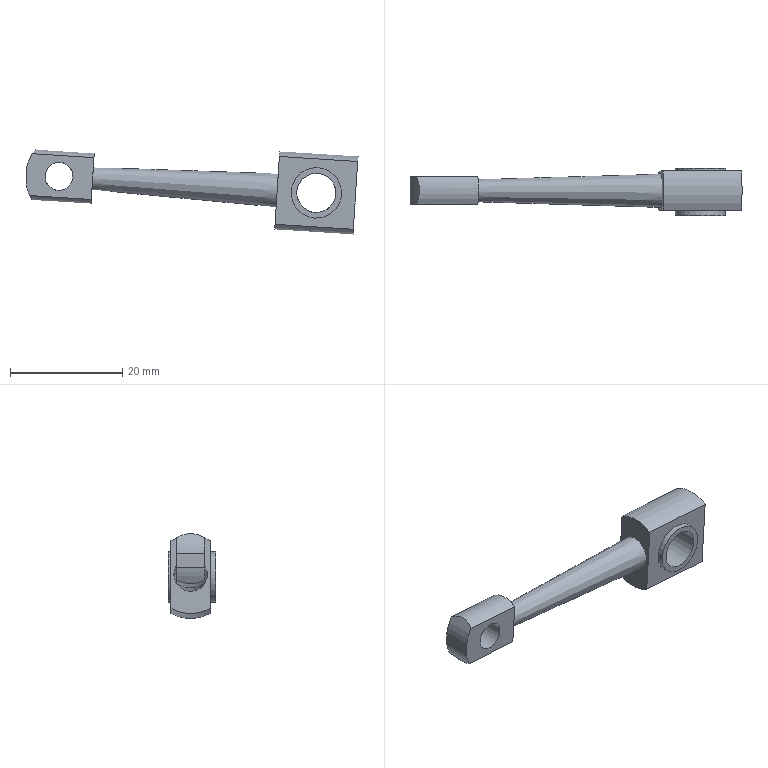Component | NX | OUTER_CASING_TUBE_CONNECTING_ROD | 1 solid | 21 faces | volume 2131 mm3 | cylinder 10 | plane 10 | cone 1 | commonest cylinder face diameters 9 x4 15 x2 14 x2 7 x1 5 x1